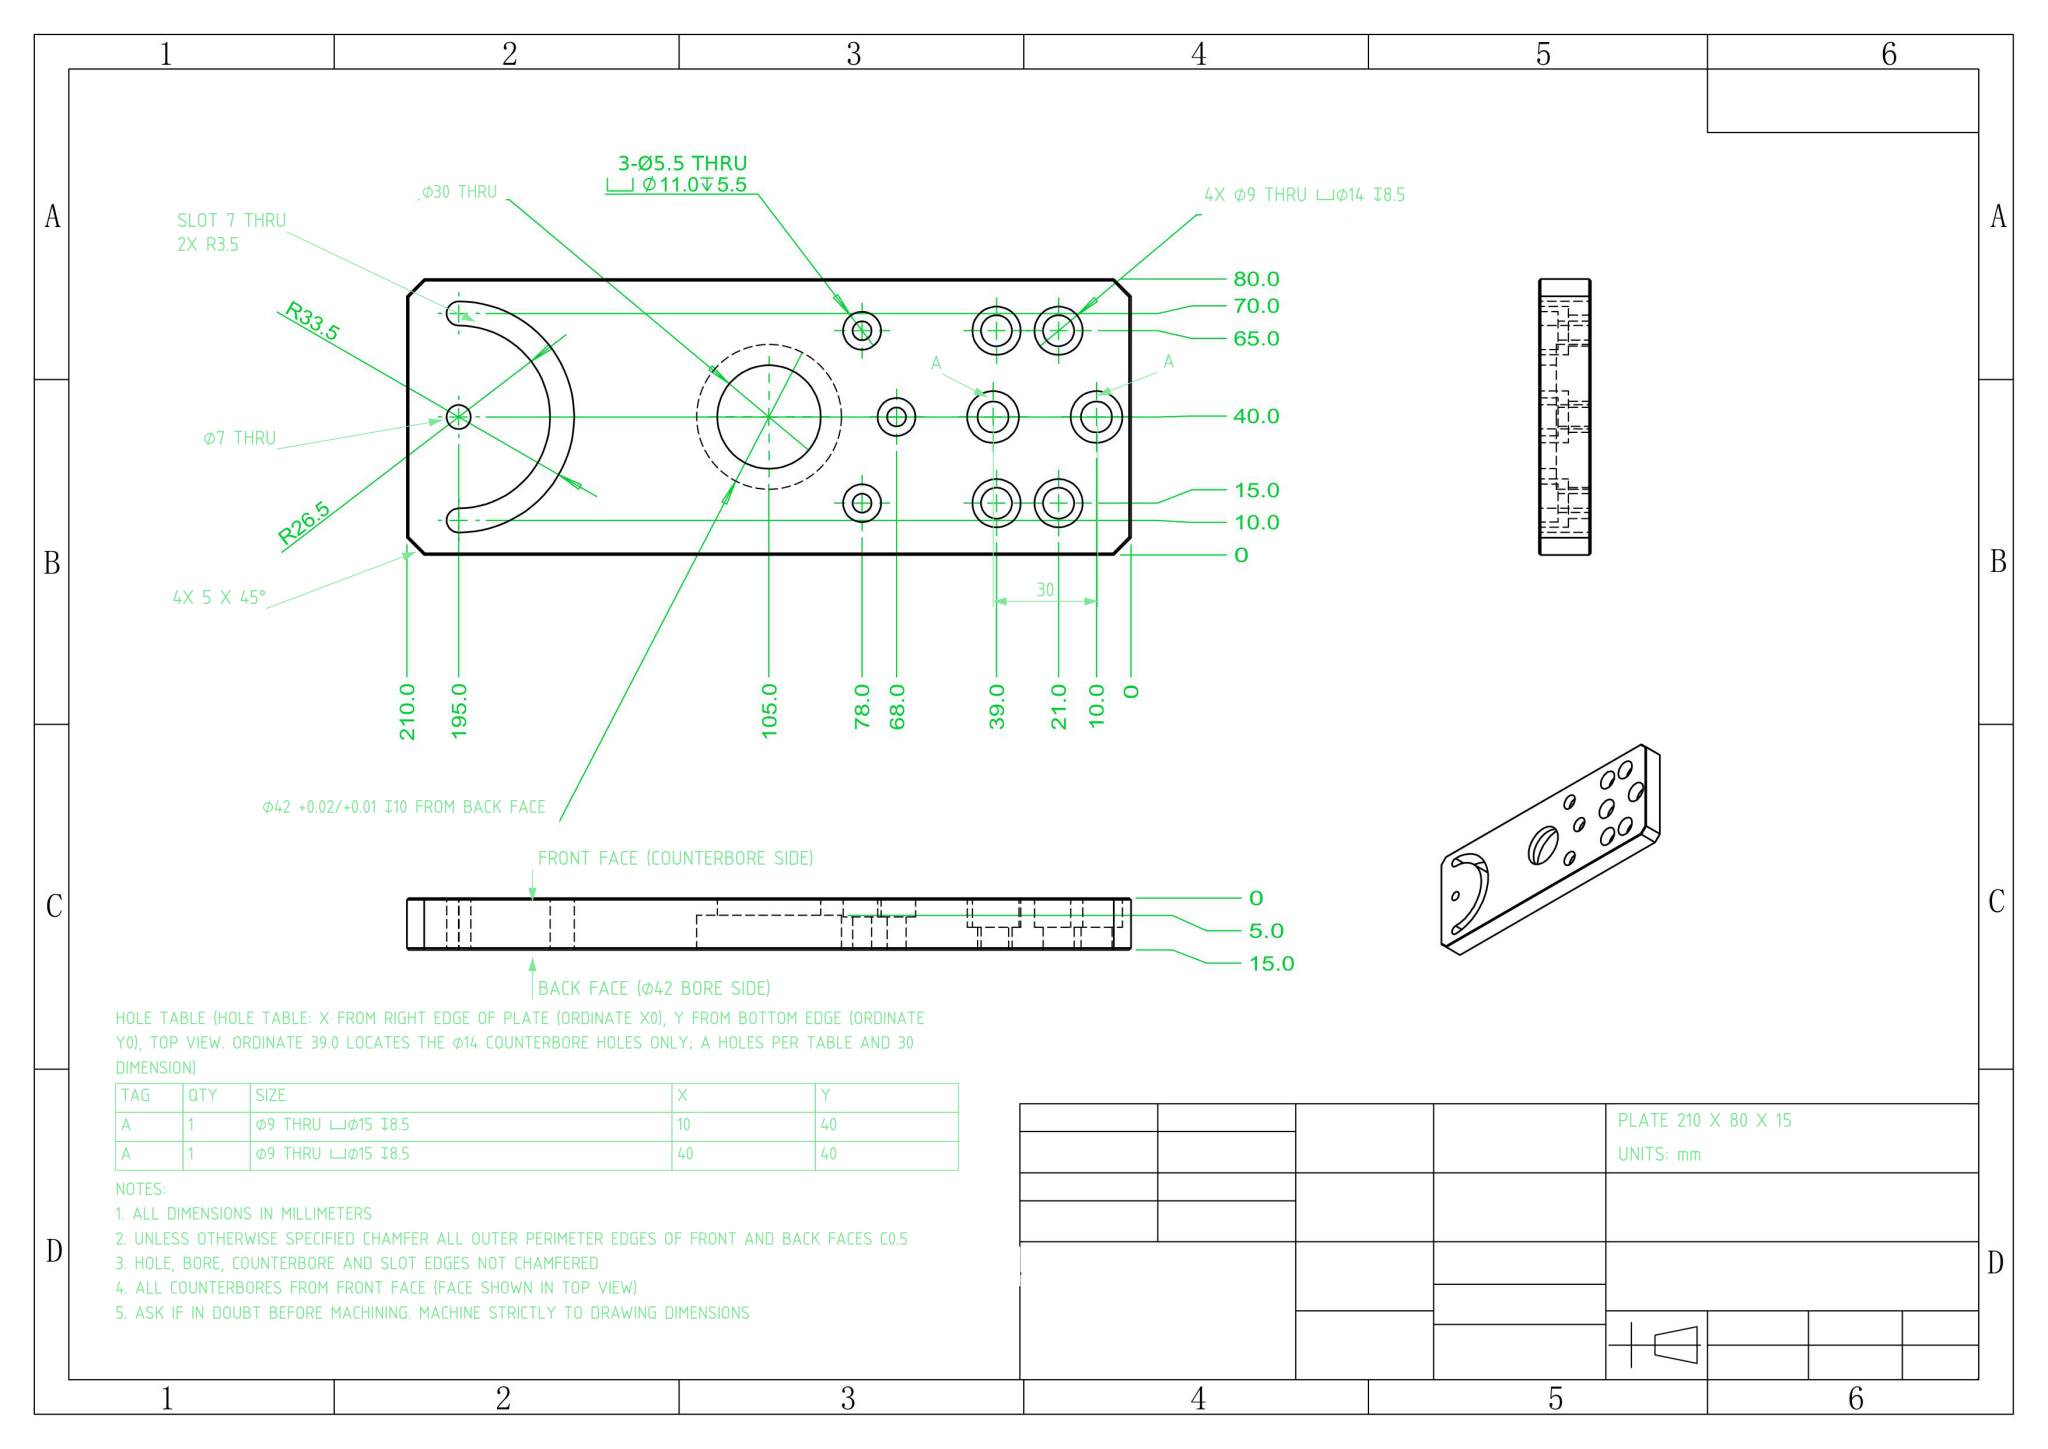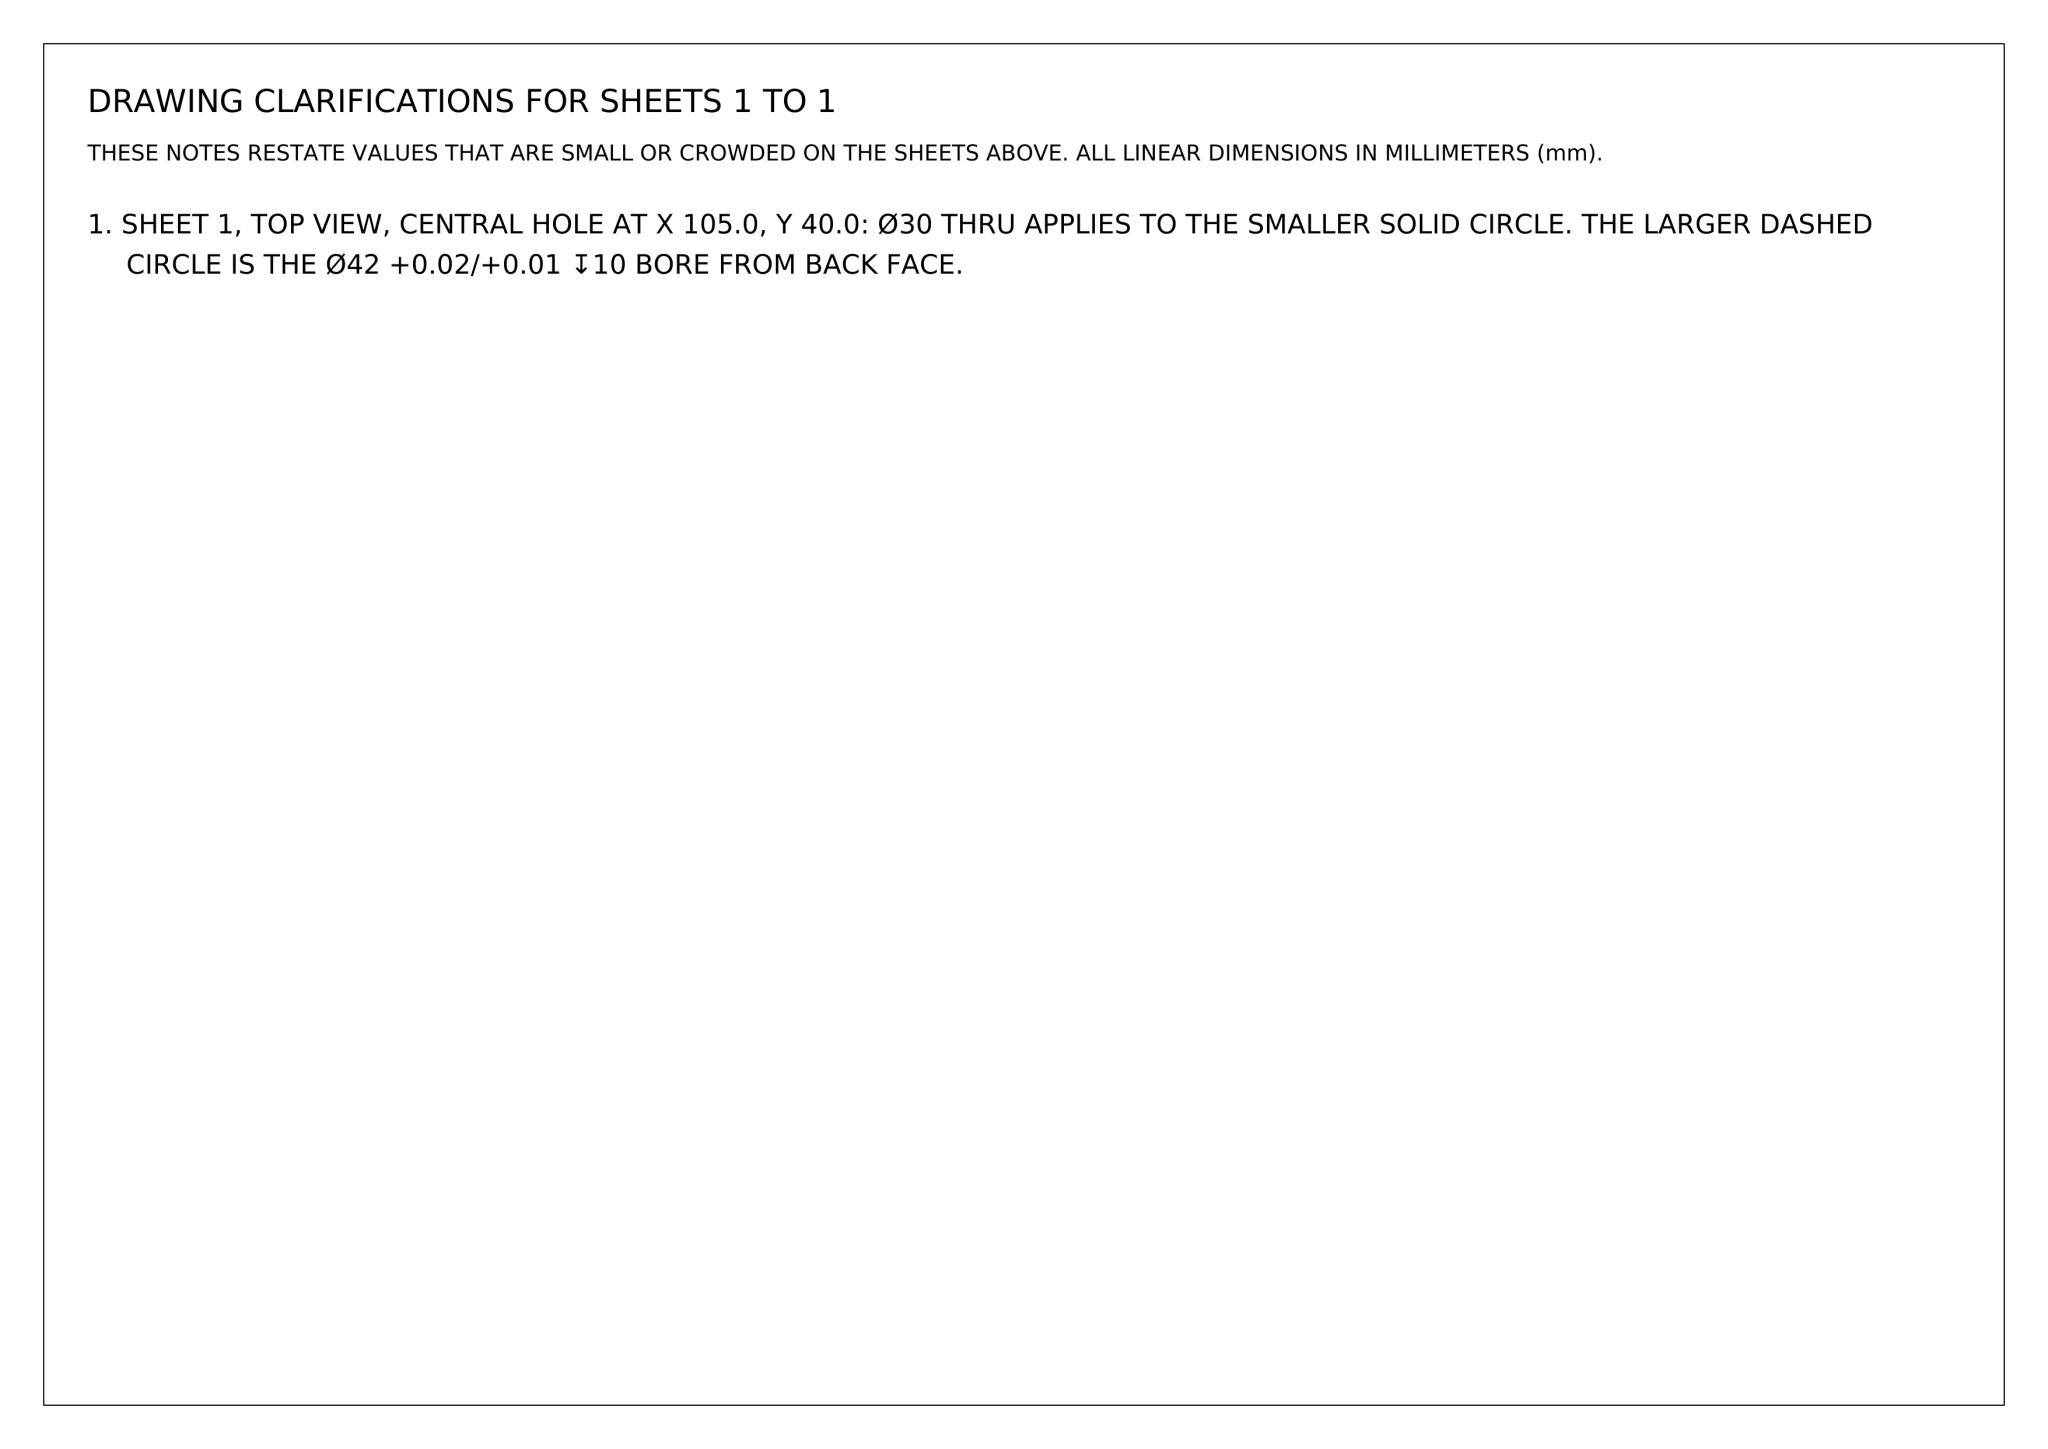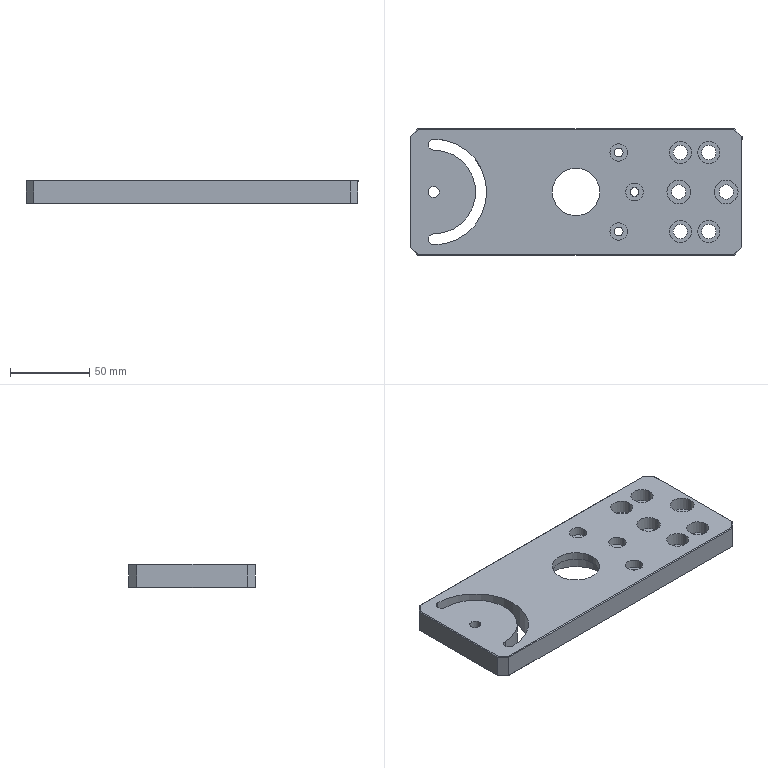Part | NX | mm | 1 solid | 84 faces | box 210 x 80 x 15 mm | volume 209705 mm3 | cylinder 48 | plane 36 | commonest cylinder face diameters 9 x12 14 x8 5.5 x6 7 x6 11 x6 15 x4 42 x2 30 x2